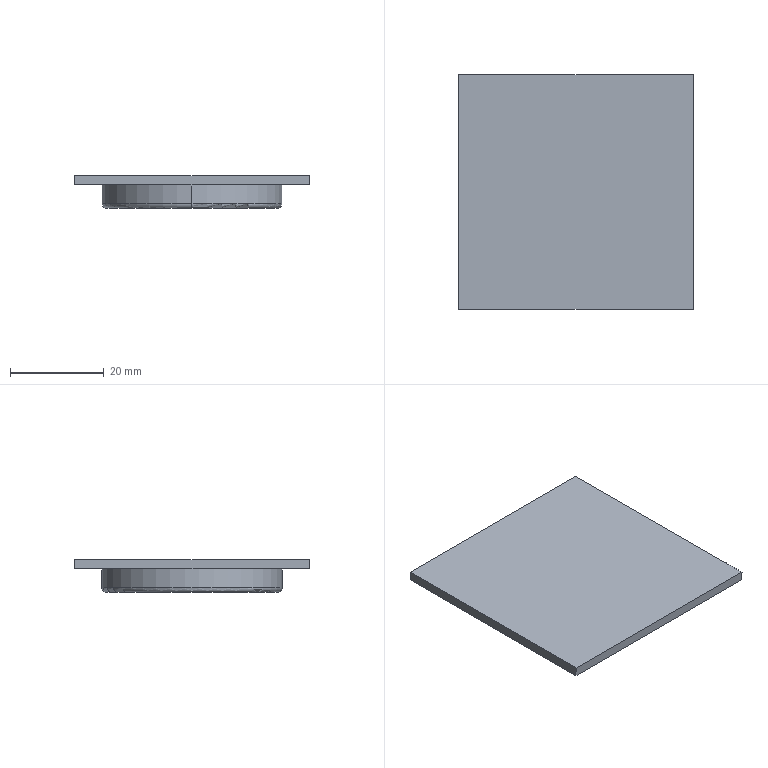Component | SolidWorks | HeightSensor-1 | 1 solid | 11 faces | box 50 x 50 x 7 mm | volume 10765 mm3 | plane 7 | torus 2 | cylinder 2 | commonest cylinder face diameters 38.4 x2
STEP:
#1=COLOUR_RGB('',0.7922,0.8196,0.9333);
#2=FILL_AREA_STYLE_COLOUR('',#1);
#3=FILL_AREA_STYLE('',(#2));
#4=SURFACE_STYLE_FILL_AREA(#3);
#5=SURFACE_SIDE_STYLE('',(#4));
#6=SURFACE_STYLE_USAGE(.BOTH.,#5);
#7=PRESENTATION_STYLE_ASSIGNMENT((#6));
#8=CARTESIAN_POINT('',(44.594,41.107,135.215));
#9=VERTEX_POINT('',#8);
#10=CARTESIAN_POINT('',(44.594,42.619,135.215));
#11=VERTEX_POINT('',#10);
#12=CARTESIAN_POINT('',(44.594,41.863,135.215));
#13=DIRECTION('',(0.,-0.,1.));
#14=DIRECTION('',(0.,1.,0.));
#15=AXIS2_PLACEMENT_3D('',#12,#13,#14);
#16=CIRCLE('',#15,0.7559);
#17=EDGE_CURVE('',#9,#11,#16,.T.);
#18=ORIENTED_EDGE('',*,*,#17,.F.);
#19=CARTESIAN_POINT('',(44.594,41.146,135.175));
#20=VERTEX_POINT('',#19);
#21=CARTESIAN_POINT('',(44.594,41.146,135.215));
#22=DIRECTION('',(1.,0.,0.));
#23=DIRECTION('',(0.,1.,0.));
#24=AXIS2_PLACEMENT_3D('',#21,#22,#23);
#25=CIRCLE('',#24,0.03937);
#26=EDGE_CURVE('',#9,#20,#25,.T.);
#27=ORIENTED_EDGE('',*,*,#26,.T.);
#28=CARTESIAN_POINT('',(44.594,42.579,135.175));
#29=VERTEX_POINT('',#28);
#30=CARTESIAN_POINT('',(44.594,41.863,135.175));
#31=DIRECTION('',(0.,0.,-1.));
#32=DIRECTION('',(0.,1.,0.));
#33=AXIS2_PLACEMENT_3D('',#30,#31,#32);
#34=CIRCLE('',#33,0.7165);
#35=EDGE_CURVE('',#29,#20,#34,.T.);
#36=ORIENTED_EDGE('',*,*,#35,.F.);
#37=CARTESIAN_POINT('',(44.594,42.579,135.215));
#38=DIRECTION('',(-1.,0.,0.));
#39=DIRECTION('',(0.,0.,1.));
#40=AXIS2_PLACEMENT_3D('',#37,#38,#39);
#41=CIRCLE('',#40,0.03937);
#42=EDGE_CURVE('',#11,#29,#41,.T.);
#43=ORIENTED_EDGE('',*,*,#42,.F.);
#44=EDGE_LOOP('',(#18,#27,#36,#43));
#45=FACE_OUTER_BOUND('',#44,.T.);
#46=CARTESIAN_POINT('',(44.594,41.863,135.215));
#47=DIRECTION('',(0.,0.,-1.));
#48=DIRECTION('',(0.,1.,0.));
#49=AXIS2_PLACEMENT_3D('',#46,#47,#48);
#50=TOROIDAL_SURFACE('',#49,0.7165,0.03937);
#51=ADVANCED_FACE('',(#45),#50,.T.);
#52=ORIENTED_EDGE('',*,*,#17,.T.);
#53=CARTESIAN_POINT('',(44.594,42.619,135.372));
#54=VERTEX_POINT('',#53);
#55=CARTESIAN_POINT('',(44.594,42.619,135.175));
#56=DIRECTION('',(0.,-0.,1.));
#57=VECTOR('',#56,39.37);
#58=LINE('',#55,#57);
#59=EDGE_CURVE('',#11,#54,#58,.T.);
#60=ORIENTED_EDGE('',*,*,#59,.T.);
#61=CARTESIAN_POINT('',(44.594,41.107,135.372));
#62=VERTEX_POINT('',#61);
#63=CARTESIAN_POINT('',(44.594,41.863,135.372));
#64=DIRECTION('',(0.,0.,-1.));
#65=DIRECTION('',(0.,1.,0.));
#66=AXIS2_PLACEMENT_3D('',#63,#64,#65);
#67=CIRCLE('',#66,0.7559);
#68=EDGE_CURVE('',#54,#62,#67,.T.);
#69=ORIENTED_EDGE('',*,*,#68,.T.);
#70=CARTESIAN_POINT('',(44.594,41.107,135.175));
#71=DIRECTION('',(0.,-0.,1.));
#72=VECTOR('',#71,39.37);
#73=LINE('',#70,#72);
#74=EDGE_CURVE('',#9,#62,#73,.T.);
#75=ORIENTED_EDGE('',*,*,#74,.F.);
#76=EDGE_LOOP('',(#52,#60,#69,#75));
#77=FACE_OUTER_BOUND('',#76,.T.);
#78=CARTESIAN_POINT('',(44.594,41.863,135.175));
#79=DIRECTION('',(0.,-0.,1.));
#80=DIRECTION('',(0.,-1.,0.));
#81=AXIS2_PLACEMENT_3D('',#78,#79,#80);
#82=CYLINDRICAL_SURFACE('',#81,0.7559);
#83=ADVANCED_FACE('',(#77),#82,.T.);
#84=CARTESIAN_POINT('',(45.578,42.847,135.372));
#85=VERTEX_POINT('',#84);
#86=CARTESIAN_POINT('',(45.578,40.878,135.372));
#87=VERTEX_POINT('',#86);
#88=CARTESIAN_POINT('',(45.578,40.878,135.372));
#89=DIRECTION('',(-0.,-1.,-0.));
#90=VECTOR('',#89,39.37);
#91=LINE('',#88,#90);
#92=EDGE_CURVE('',#85,#87,#91,.T.);
#93=ORIENTED_EDGE('',*,*,#92,.F.);
#94=CARTESIAN_POINT('',(45.578,42.847,135.451));
#95=VERTEX_POINT('',#94);
#96=CARTESIAN_POINT('',(45.578,42.847,135.451));
#97=DIRECTION('',(0.,0.,-1.));
#98=VECTOR('',#97,39.37);
#99=LINE('',#96,#98);
#100=EDGE_CURVE('',#95,#85,#99,.T.);
#101=ORIENTED_EDGE('',*,*,#100,.F.);
#102=CARTESIAN_POINT('',(45.578,40.878,135.451));
#103=VERTEX_POINT('',#102);
#104=CARTESIAN_POINT('',(45.578,40.878,135.451));
#105=DIRECTION('',(-0.,-1.,-0.));
#106=VECTOR('',#105,39.37);
#107=LINE('',#104,#106);
#108=EDGE_CURVE('',#95,#103,#107,.T.);
#109=ORIENTED_EDGE('',*,*,#108,.T.);
#110=CARTESIAN_POINT('',(45.578,40.878,135.451));
#111=DIRECTION('',(0.,0.,-1.));
#112=VECTOR('',#111,39.37);
#113=LINE('',#110,#112);
#114=EDGE_CURVE('',#103,#87,#113,.T.);
#115=ORIENTED_EDGE('',*,*,#114,.T.);
#116=EDGE_LOOP('',(#93,#101,#109,#115));
#117=FACE_OUTER_BOUND('',#116,.T.);
#118=CARTESIAN_POINT('',(45.578,40.878,135.451));
#119=DIRECTION('',(1.,-0.,-0.));
#120=DIRECTION('',(-0.,-1.,-0.));
#121=AXIS2_PLACEMENT_3D('',#118,#119,#120);
#122=PLANE('',#121);
#123=ADVANCED_FACE('',(#117),#122,.T.);
#124=CARTESIAN_POINT('',(43.61,42.847,135.372));
#125=VERTEX_POINT('',#124);
#126=CARTESIAN_POINT('',(43.61,42.847,135.372));
#127=DIRECTION('',(1.,0.,0.));
#128=VECTOR('',#127,39.37);
#129=LINE('',#126,#128);
#130=EDGE_CURVE('',#125,#85,#129,.T.);
#131=ORIENTED_EDGE('',*,*,#130,.F.);
#132=CARTESIAN_POINT('',(43.61,42.847,135.451));
#133=VERTEX_POINT('',#132);
#134=CARTESIAN_POINT('',(43.61,42.847,135.451));
#135=DIRECTION('',(0.,0.,-1.));
#136=VECTOR('',#135,39.37);
#137=LINE('',#134,#136);
#138=EDGE_CURVE('',#133,#125,#137,.T.);
#139=ORIENTED_EDGE('',*,*,#138,.F.);
#140=CARTESIAN_POINT('',(43.61,42.847,135.451));
#141=DIRECTION('',(1.,0.,0.));
#142=VECTOR('',#141,39.37);
#143=LINE('',#140,#142);
#144=EDGE_CURVE('',#133,#95,#143,.T.);
#145=ORIENTED_EDGE('',*,*,#144,.T.);
#146=ORIENTED_EDGE('',*,*,#100,.T.);
#147=EDGE_LOOP('',(#131,#139,#145,#146));
#148=FACE_OUTER_BOUND('',#147,.T.);
#149=CARTESIAN_POINT('',(43.61,42.847,135.451));
#150=DIRECTION('',(0.,1.,0.));
#151=DIRECTION('',(1.,0.,0.));
#152=AXIS2_PLACEMENT_3D('',#149,#150,#151);
#153=PLANE('',#152);
#154=ADVANCED_FACE('',(#148),#153,.T.);
#155=CARTESIAN_POINT('',(43.61,40.878,135.372));
#156=VERTEX_POINT('',#155);
#157=CARTESIAN_POINT('',(43.61,40.878,135.372));
#158=DIRECTION('',(0.,1.,0.));
#159=VECTOR('',#158,39.37);
#160=LINE('',#157,#159);
#161=EDGE_CURVE('',#156,#125,#160,.T.);
#162=ORIENTED_EDGE('',*,*,#161,.F.);
#163=CARTESIAN_POINT('',(43.61,40.878,135.451));
#164=VERTEX_POINT('',#163);
#165=CARTESIAN_POINT('',(43.61,40.878,135.451));
#166=DIRECTION('',(0.,0.,-1.));
#167=VECTOR('',#166,39.37);
#168=LINE('',#165,#167);
#169=EDGE_CURVE('',#164,#156,#168,.T.);
#170=ORIENTED_EDGE('',*,*,#169,.F.);
#171=CARTESIAN_POINT('',(43.61,40.878,135.451));
#172=DIRECTION('',(0.,1.,0.));
#173=VECTOR('',#172,39.37);
#174=LINE('',#171,#173);
#175=EDGE_CURVE('',#164,#133,#174,.T.);
#176=ORIENTED_EDGE('',*,*,#175,.T.);
#177=ORIENTED_EDGE('',*,*,#138,.T.);
#178=EDGE_LOOP('',(#162,#170,#176,#177));
#179=FACE_OUTER_BOUND('',#178,.T.);
#180=CARTESIAN_POINT('',(43.61,40.878,135.451));
#181=DIRECTION('',(-1.,0.,0.));
#182=DIRECTION('',(0.,1.,0.));
#183=AXIS2_PLACEMENT_3D('',#180,#181,#182);
#184=PLANE('',#183);
#185=ADVANCED_FACE('',(#179),#184,.T.);
#186=CARTESIAN_POINT('',(43.61,40.878,135.372));
#187=DIRECTION('',(-1.,0.,0.));
#188=VECTOR('',#187,39.37);
#189=LINE('',#186,#188);
#190=EDGE_CURVE('',#87,#156,#189,.T.);
#191=ORIENTED_EDGE('',*,*,#190,.F.);
#192=ORIENTED_EDGE('',*,*,#114,.F.);
#193=CARTESIAN_POINT('',(43.61,40.878,135.451));
#194=DIRECTION('',(-1.,0.,0.));
#195=VECTOR('',#194,39.37);
#196=LINE('',#193,#195);
#197=EDGE_CURVE('',#103,#164,#196,.T.);
#198=ORIENTED_EDGE('',*,*,#197,.T.);
#199=ORIENTED_EDGE('',*,*,#169,.T.);
#200=EDGE_LOOP('',(#191,#192,#198,#199));
#201=FACE_OUTER_BOUND('',#200,.T.);
#202=CARTESIAN_POINT('',(43.61,40.878,135.451));
#203=DIRECTION('',(0.,-1.,-0.));
#204=DIRECTION('',(-1.,0.,0.));
#205=AXIS2_PLACEMENT_3D('',#202,#203,#204);
#206=PLANE('',#205);
#207=ADVANCED_FACE('',(#201),#206,.T.);
#208=ORIENTED_EDGE('',*,*,#108,.F.);
#209=ORIENTED_EDGE('',*,*,#144,.F.);
#210=ORIENTED_EDGE('',*,*,#175,.F.);
#211=ORIENTED_EDGE('',*,*,#197,.F.);
#212=EDGE_LOOP('',(#208,#209,#210,#211));
#213=FACE_OUTER_BOUND('',#212,.T.);
#214=CARTESIAN_POINT('',(44.594,41.863,135.451));
#215=DIRECTION('',(0.,0.,-1.));
#216=DIRECTION('',(0.,1.,0.));
#217=AXIS2_PLACEMENT_3D('',#214,#215,#216);
#218=PLANE('',#217);
#219=ADVANCED_FACE('',(#213),#218,.F.);
#220=CARTESIAN_POINT('',(44.594,41.863,135.372));
#221=DIRECTION('',(0.,0.,-1.));
#222=DIRECTION('',(0.,1.,0.));
#223=AXIS2_PLACEMENT_3D('',#220,#221,#222);
#224=CIRCLE('',#223,0.7559);
#225=EDGE_CURVE('',#62,#54,#224,.T.);
#226=ORIENTED_EDGE('',*,*,#225,.F.);
#227=ORIENTED_EDGE('',*,*,#68,.F.);
#228=EDGE_LOOP('',(#226,#227));
#229=FACE_BOUND('',#228,.T.);
#230=ORIENTED_EDGE('',*,*,#92,.T.);
#231=ORIENTED_EDGE('',*,*,#190,.T.);
#232=ORIENTED_EDGE('',*,*,#161,.T.);
#233=ORIENTED_EDGE('',*,*,#130,.T.);
#234=EDGE_LOOP('',(#230,#231,#232,#233));
#235=FACE_OUTER_BOUND('',#234,.T.);
#236=CARTESIAN_POINT('',(44.594,41.863,135.372));
#237=DIRECTION('',(0.,0.,-1.));
#238=DIRECTION('',(0.,1.,0.));
#239=AXIS2_PLACEMENT_3D('',#236,#237,#238);
#240=PLANE('',#239);
#241=ADVANCED_FACE('',(#229,#235),#240,.T.);
#242=ORIENTED_EDGE('',*,*,#59,.F.);
#243=CARTESIAN_POINT('',(44.594,41.863,135.215));
#244=DIRECTION('',(0.,-0.,1.));
#245=DIRECTION('',(0.,1.,0.));
#246=AXIS2_PLACEMENT_3D('',#243,#244,#245);
#247=CIRCLE('',#246,0.7559);
#248=EDGE_CURVE('',#11,#9,#247,.T.);
#249=ORIENTED_EDGE('',*,*,#248,.T.);
#250=ORIENTED_EDGE('',*,*,#74,.T.);
#251=ORIENTED_EDGE('',*,*,#225,.T.);
#252=EDGE_LOOP('',(#242,#249,#250,#251));
#253=FACE_OUTER_BOUND('',#252,.T.);
#254=CARTESIAN_POINT('',(44.594,41.863,135.175));
#255=DIRECTION('',(0.,-0.,1.));
#256=DIRECTION('',(0.,-1.,0.));
#257=AXIS2_PLACEMENT_3D('',#254,#255,#256);
#258=CYLINDRICAL_SURFACE('',#257,0.7559);
#259=ADVANCED_FACE('',(#253),#258,.T.);
#260=ORIENTED_EDGE('',*,*,#35,.T.);
#261=CARTESIAN_POINT('',(44.594,41.863,135.175));
#262=DIRECTION('',(0.,0.,-1.));
#263=DIRECTION('',(0.,1.,0.));
#264=AXIS2_PLACEMENT_3D('',#261,#262,#263);
#265=CIRCLE('',#264,0.7165);
#266=EDGE_CURVE('',#20,#29,#265,.T.);
#267=ORIENTED_EDGE('',*,*,#266,.T.);
#268=EDGE_LOOP('',(#260,#267));
#269=FACE_OUTER_BOUND('',#268,.T.);
#270=CARTESIAN_POINT('',(44.594,41.863,135.175));
#271=DIRECTION('',(0.,0.,-1.));
#272=DIRECTION('',(0.,1.,0.));
#273=AXIS2_PLACEMENT_3D('',#270,#271,#272);
#274=PLANE('',#273);
#275=ADVANCED_FACE('',(#269),#274,.T.);
#276=ORIENTED_EDGE('',*,*,#26,.F.);
#277=ORIENTED_EDGE('',*,*,#248,.F.);
#278=ORIENTED_EDGE('',*,*,#42,.T.);
#279=ORIENTED_EDGE('',*,*,#266,.F.);
#280=EDGE_LOOP('',(#276,#277,#278,#279));
#281=FACE_OUTER_BOUND('',#280,.T.);
#282=CARTESIAN_POINT('',(44.594,41.863,135.215));
#283=DIRECTION('',(0.,0.,-1.));
#284=DIRECTION('',(0.,1.,0.));
#285=AXIS2_PLACEMENT_3D('',#282,#283,#284);
#286=TOROIDAL_SURFACE('',#285,0.7165,0.03937);
#287=ADVANCED_FACE('',(#281),#286,.T.);
#288=CLOSED_SHELL('',(#51,#83,#123,#154,#185,#207,#219,#241,#259,#275,#287));
#289=MANIFOLD_SOLID_BREP('',#288);
#290=STYLED_ITEM('',(#7),#289);
#291=PRESENTATION_LAYER_ASSIGNMENT('','',(#290));
#292=(LENGTH_UNIT()NAMED_UNIT(*)SI_UNIT($,.METRE.));
#293=LENGTH_MEASURE_WITH_UNIT(LENGTH_MEASURE(0.0254),#292);
#294=DIMENSIONAL_EXPONENTS(1.,0.,0.,0.,0.,0.,0.);
#295=(CONVERSION_BASED_UNIT('',#293)LENGTH_UNIT()NAMED_UNIT(#294));
#296=UNCERTAINTY_MEASURE_WITH_UNIT(LENGTH_MEASURE(0.00001),#295,'','');
#297=(NAMED_UNIT(*)PLANE_ANGLE_UNIT()SI_UNIT($,.RADIAN.));
#298=(NAMED_UNIT(*)SI_UNIT($,.STERADIAN.)SOLID_ANGLE_UNIT());
#299=(GEOMETRIC_REPRESENTATION_CONTEXT(3)GLOBAL_UNCERTAINTY_ASSIGNED_CONTEXT((#296))GLOBAL_UNIT_ASSIGNED_CONTEXT((#295,#297,#298))REPRESENTATION_CONTEXT('',''));
#300=MECHANICAL_DESIGN_GEOMETRIC_PRESENTATION_REPRESENTATION('',(#290),#299);
#301=CARTESIAN_POINT('',(0.,0.,0.));
#302=DIRECTION('',(0.,0.,1.));
#303=DIRECTION('',(1.,0.,0.));
#304=AXIS2_PLACEMENT_3D('',#301,#302,#303);
#305=(LENGTH_UNIT()NAMED_UNIT(*)SI_UNIT($,.METRE.));
#306=LENGTH_MEASURE_WITH_UNIT(LENGTH_MEASURE(0.0254),#305);
#307=DIMENSIONAL_EXPONENTS(1.,0.,0.,0.,0.,0.,0.);
#308=(CONVERSION_BASED_UNIT('',#306)LENGTH_UNIT()NAMED_UNIT(#307));
#309=UNCERTAINTY_MEASURE_WITH_UNIT(LENGTH_MEASURE(0.00001),#308,'','');
#310=(NAMED_UNIT(*)PLANE_ANGLE_UNIT()SI_UNIT($,.RADIAN.));
#311=(NAMED_UNIT(*)SI_UNIT($,.STERADIAN.)SOLID_ANGLE_UNIT());
#312=(GEOMETRIC_REPRESENTATION_CONTEXT(3)GLOBAL_UNCERTAINTY_ASSIGNED_CONTEXT((#309))GLOBAL_UNIT_ASSIGNED_CONTEXT((#308,#310,#311))REPRESENTATION_CONTEXT('',''));
#313=ADVANCED_BREP_SHAPE_REPRESENTATION('',(#289,#304),#312);